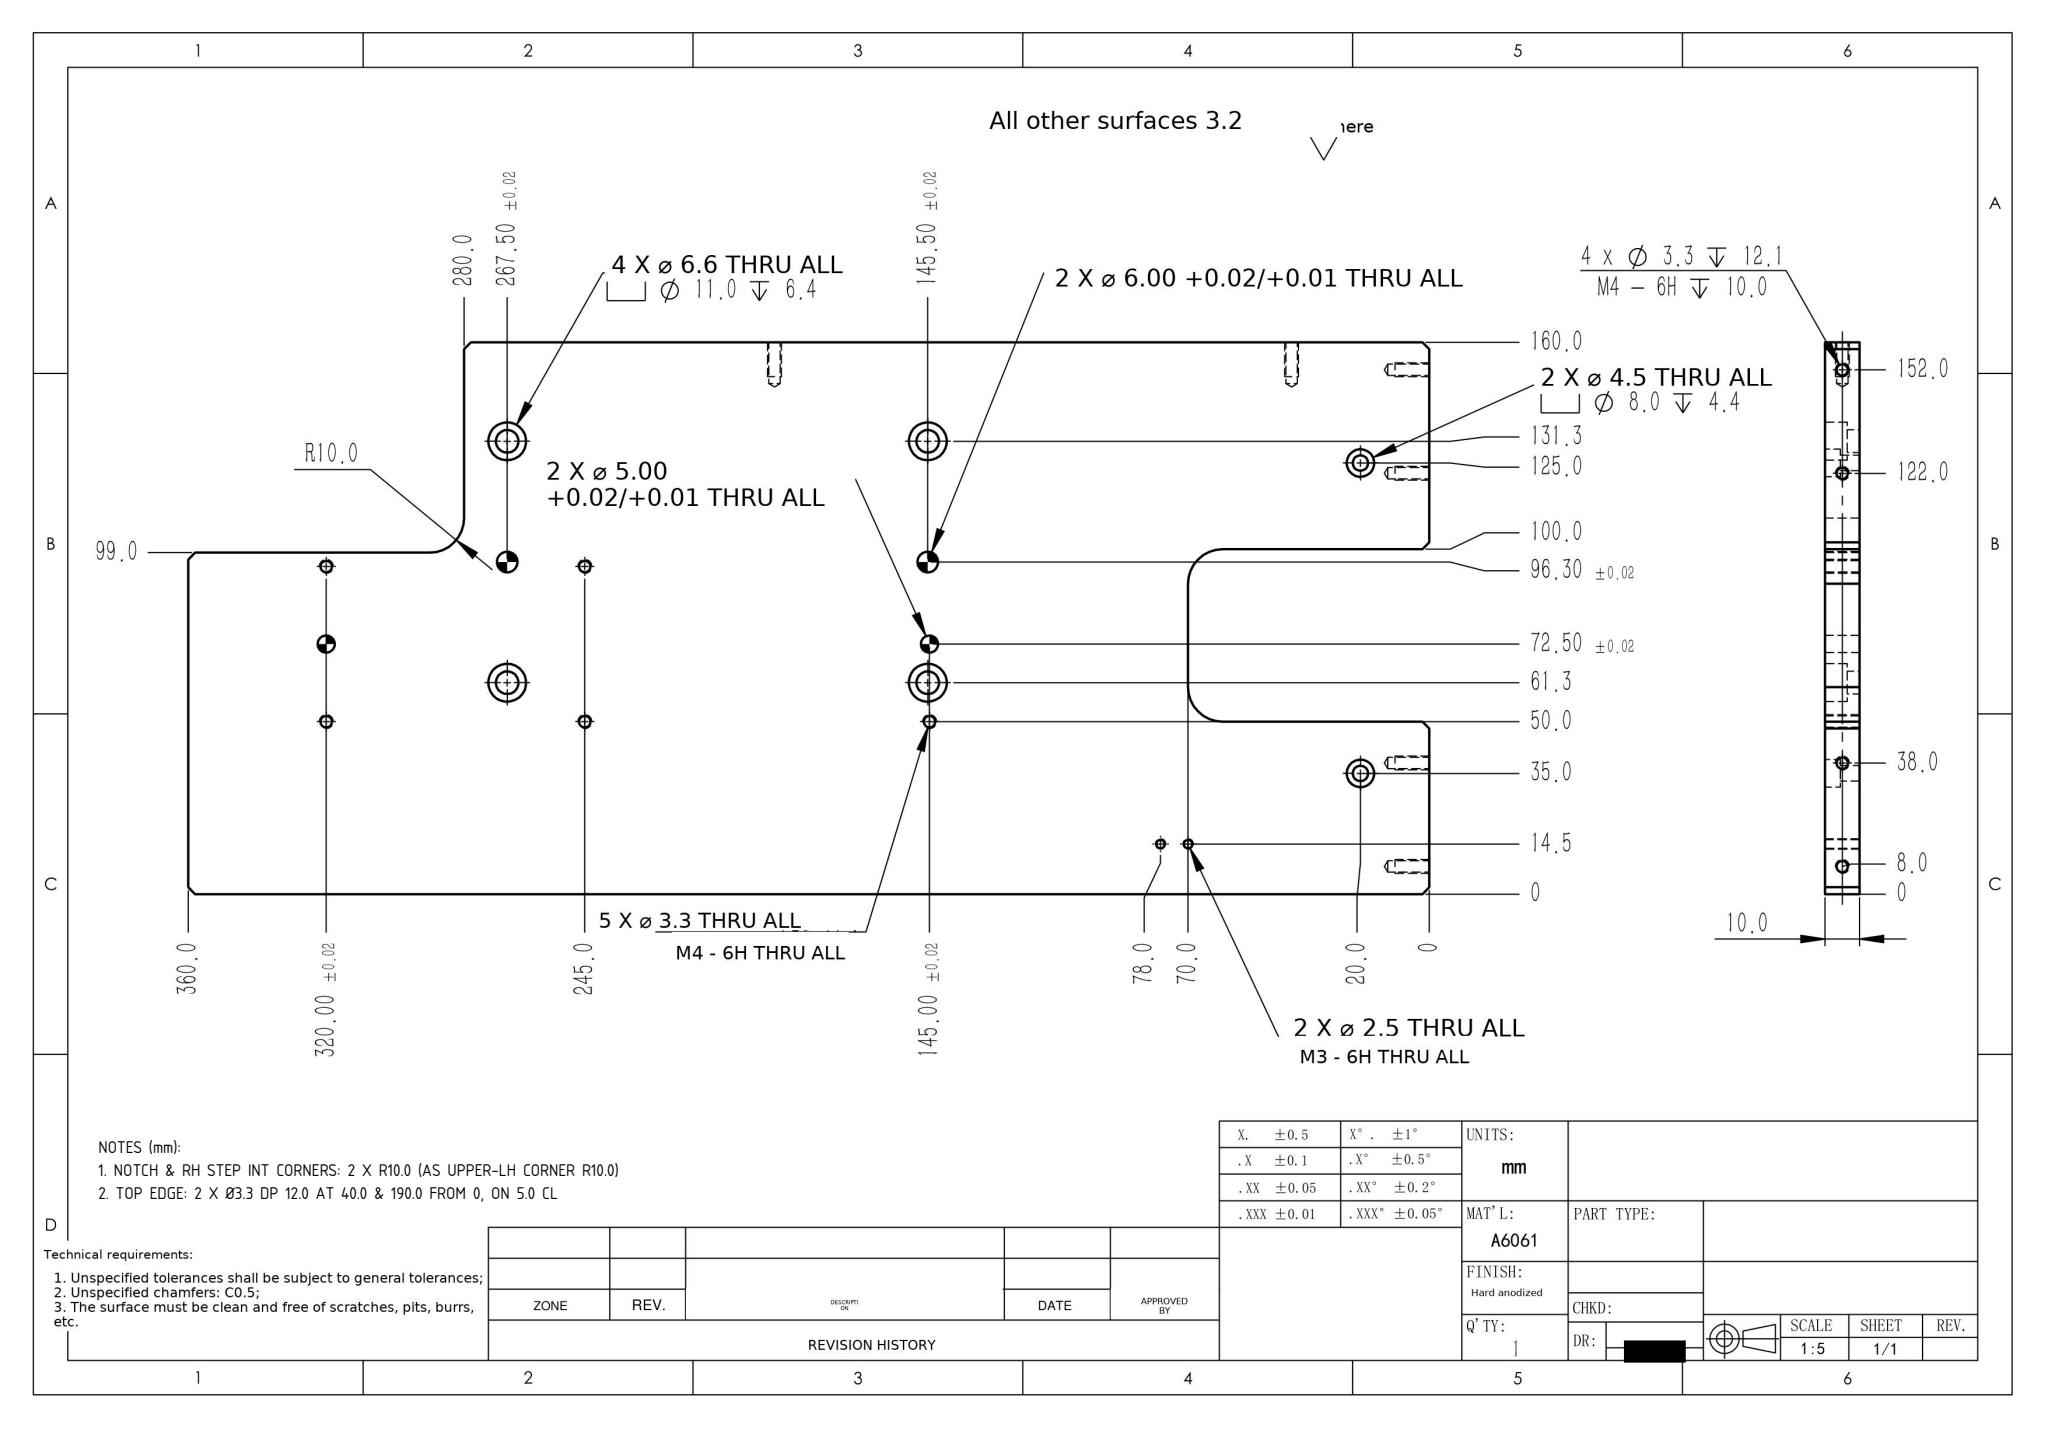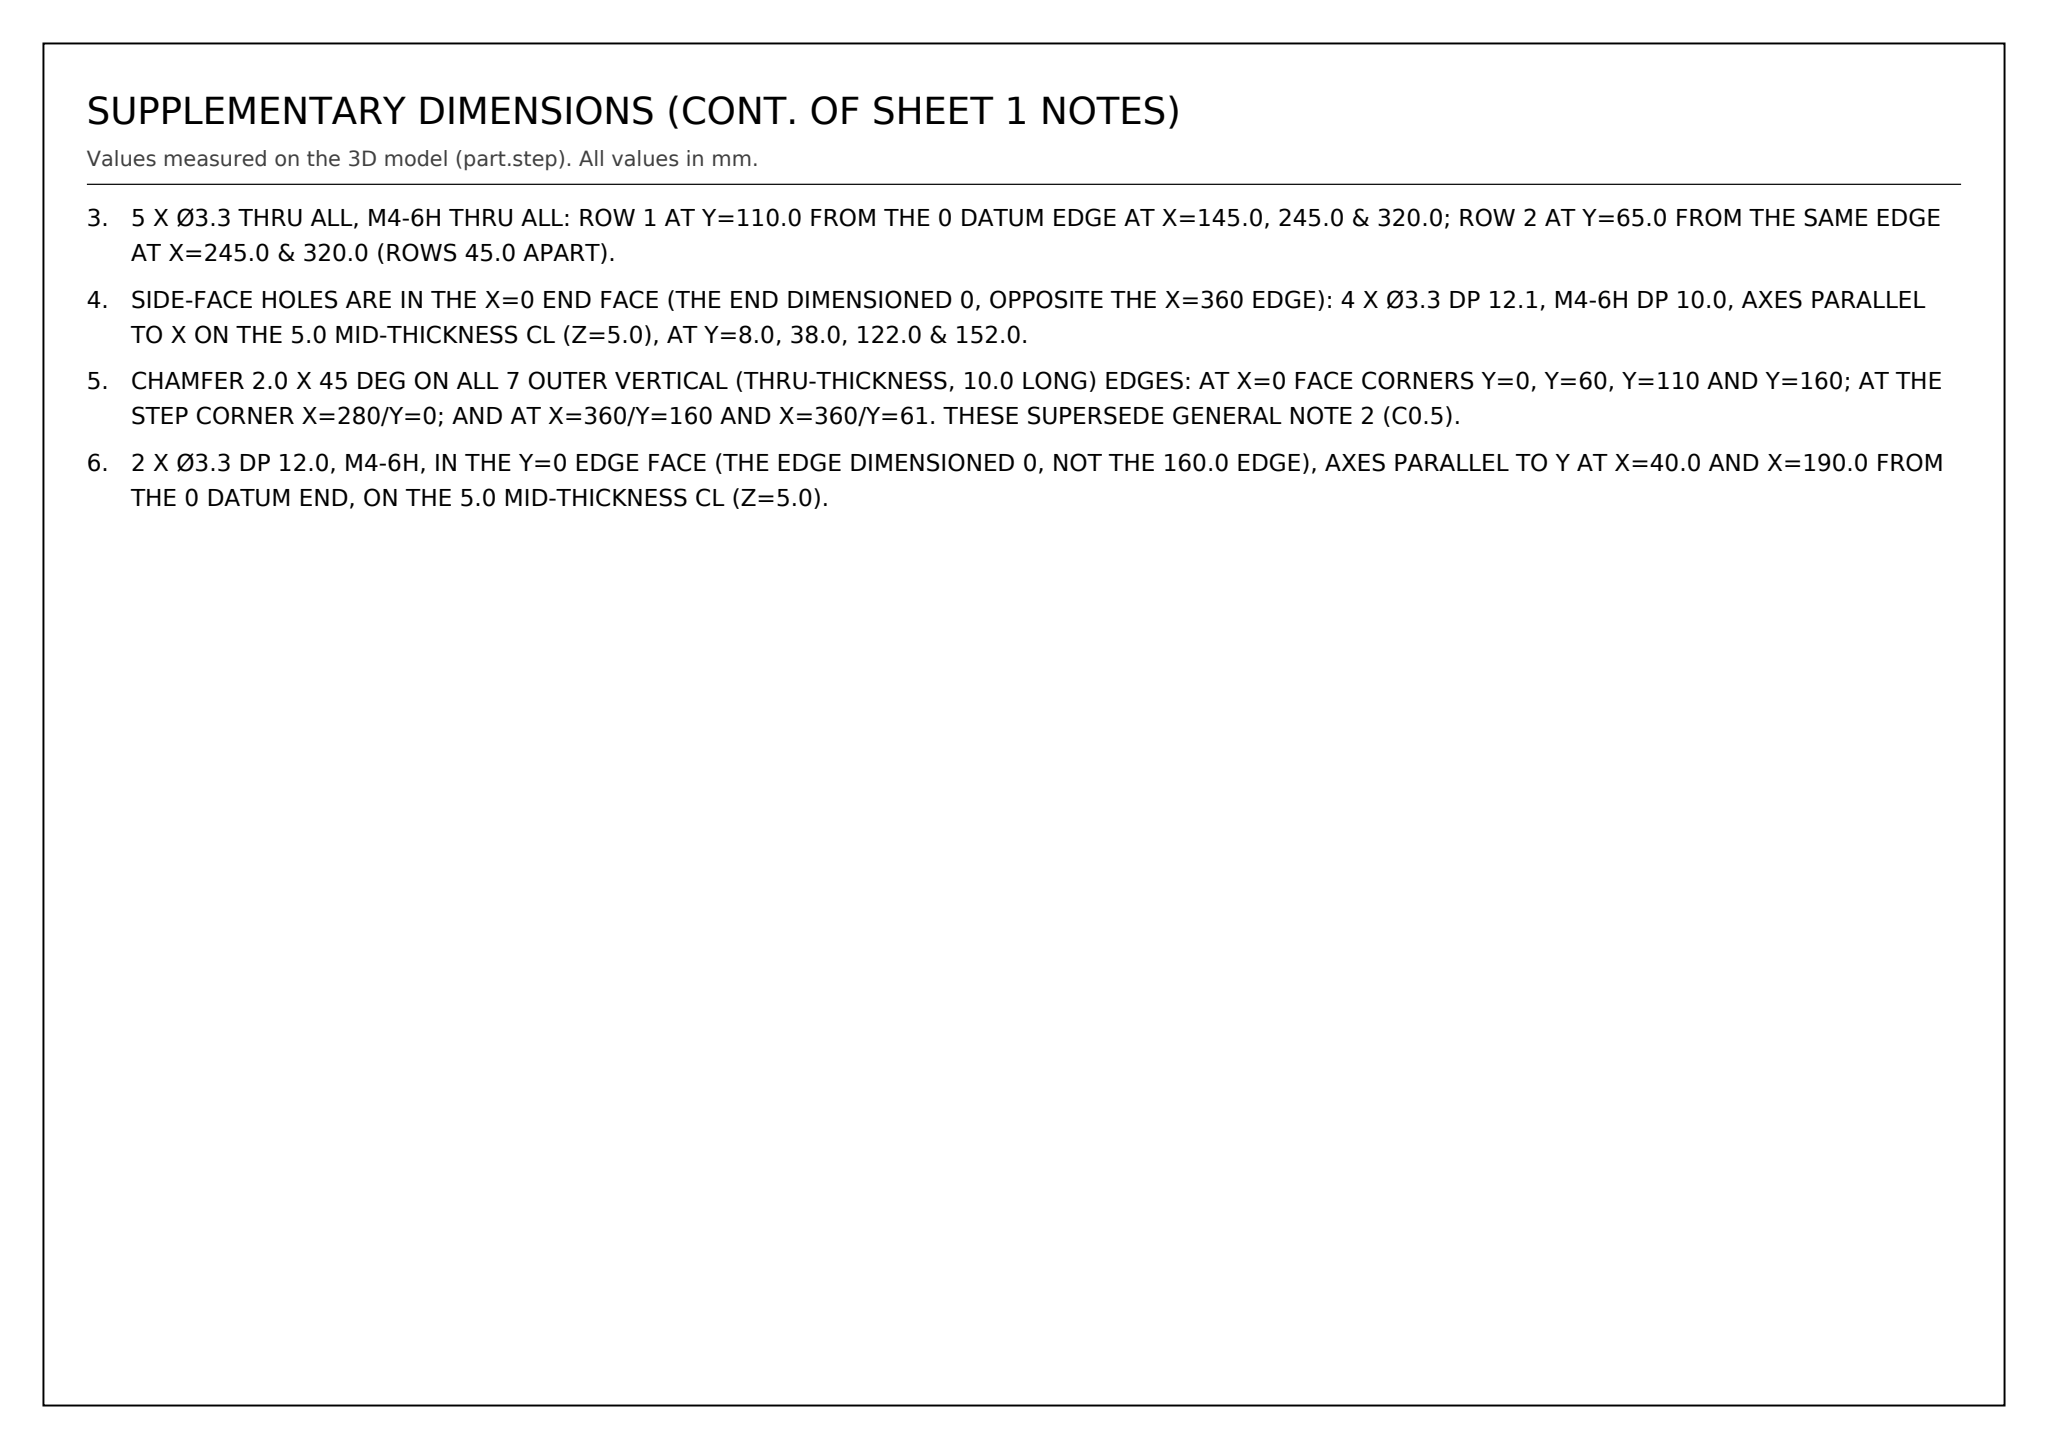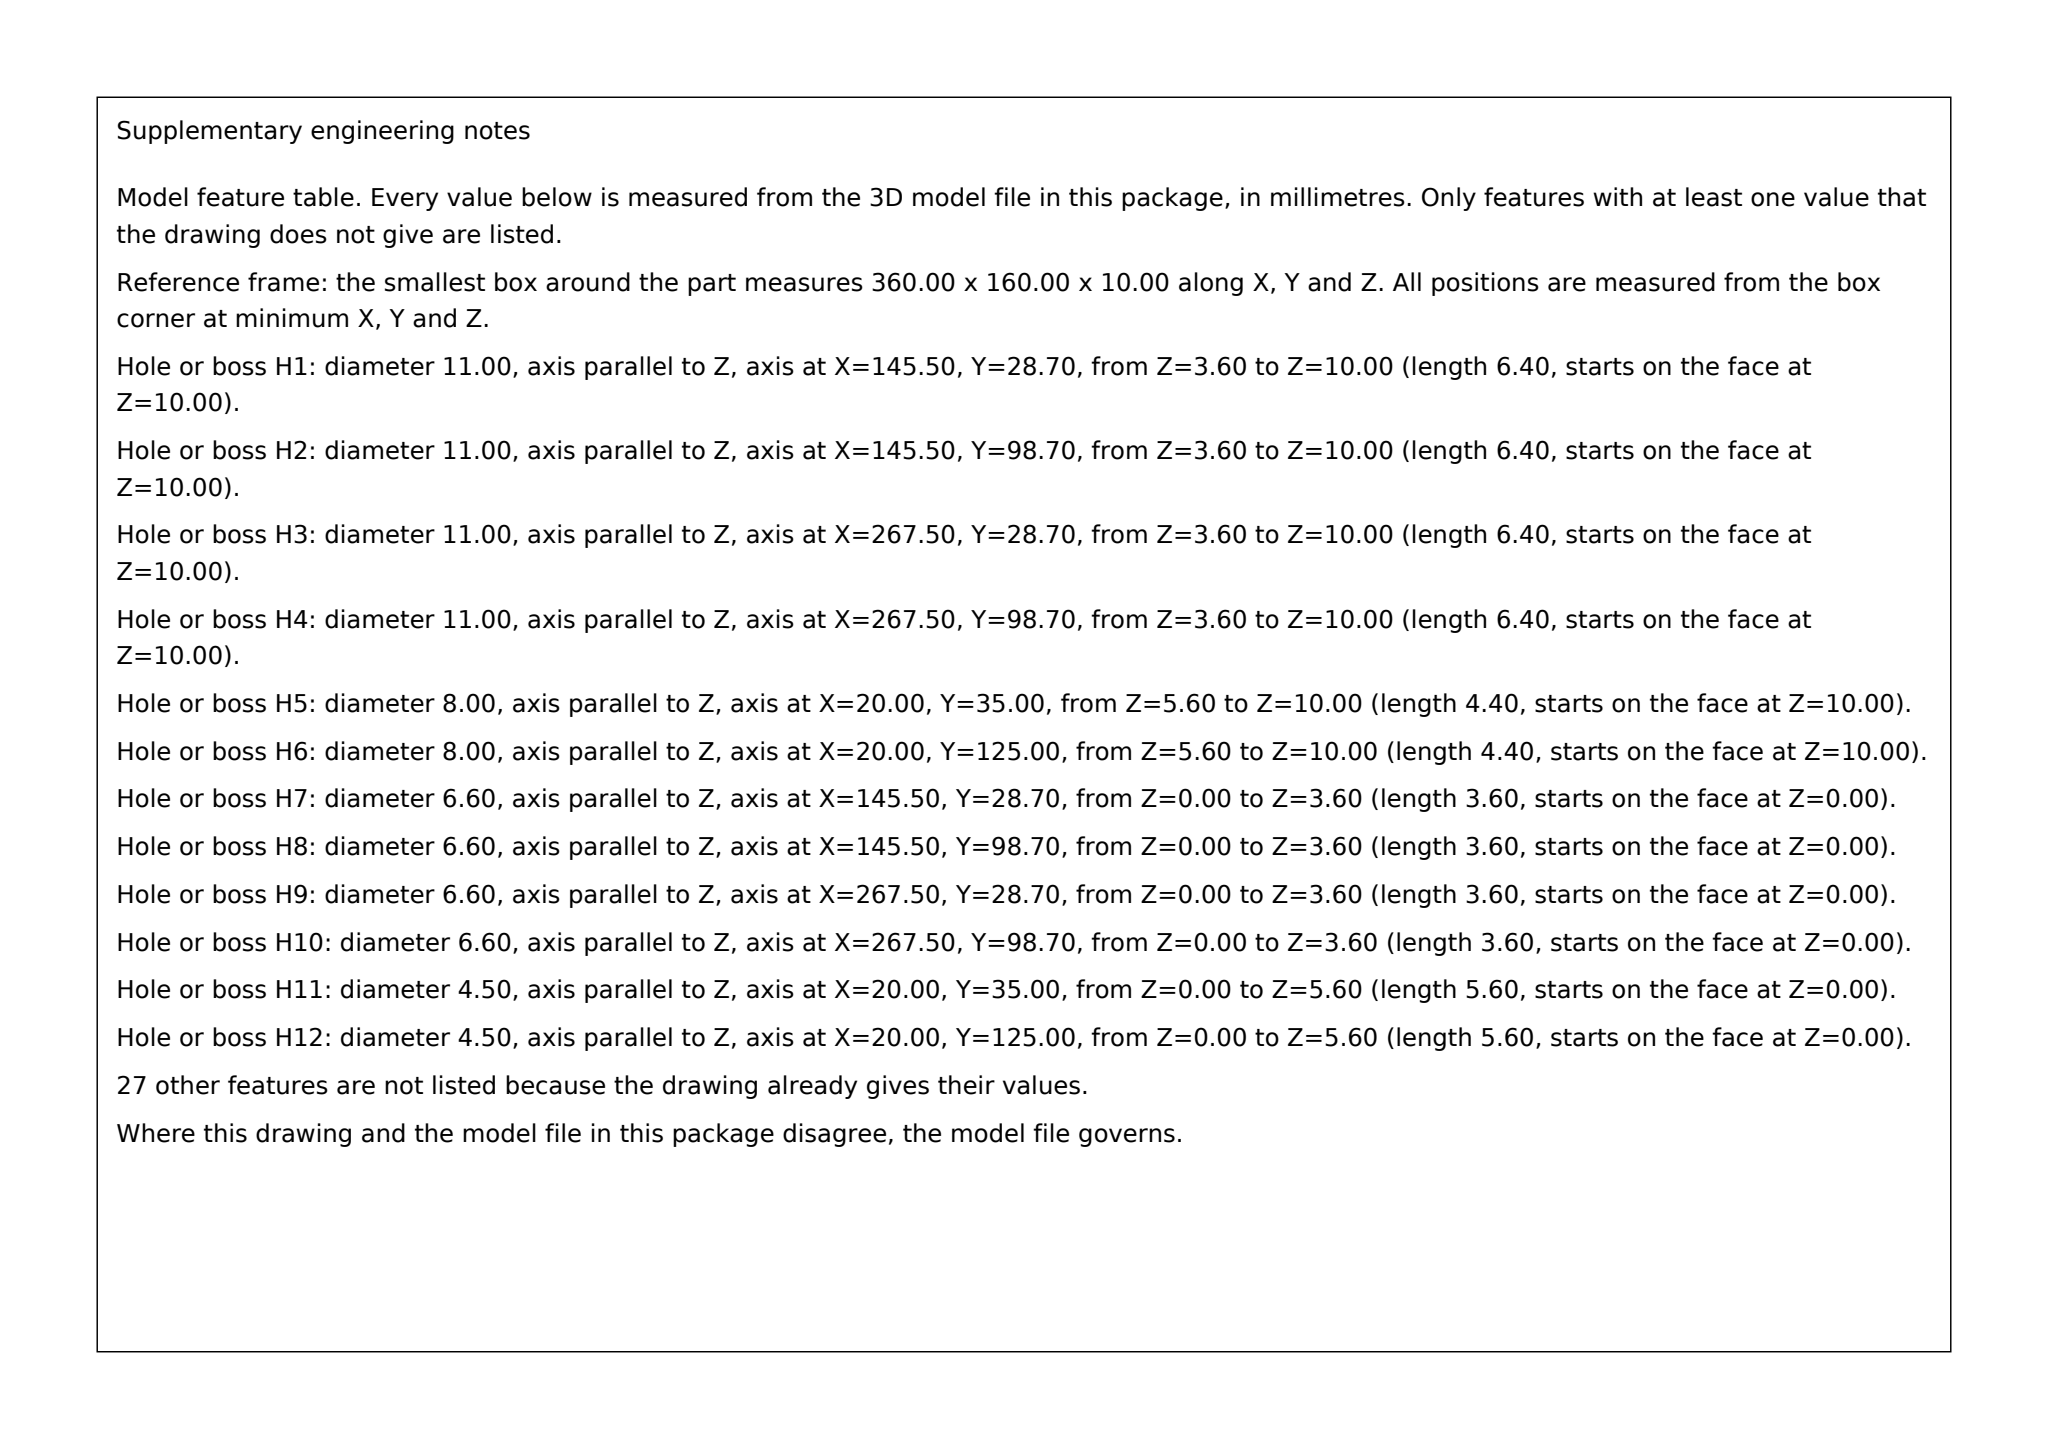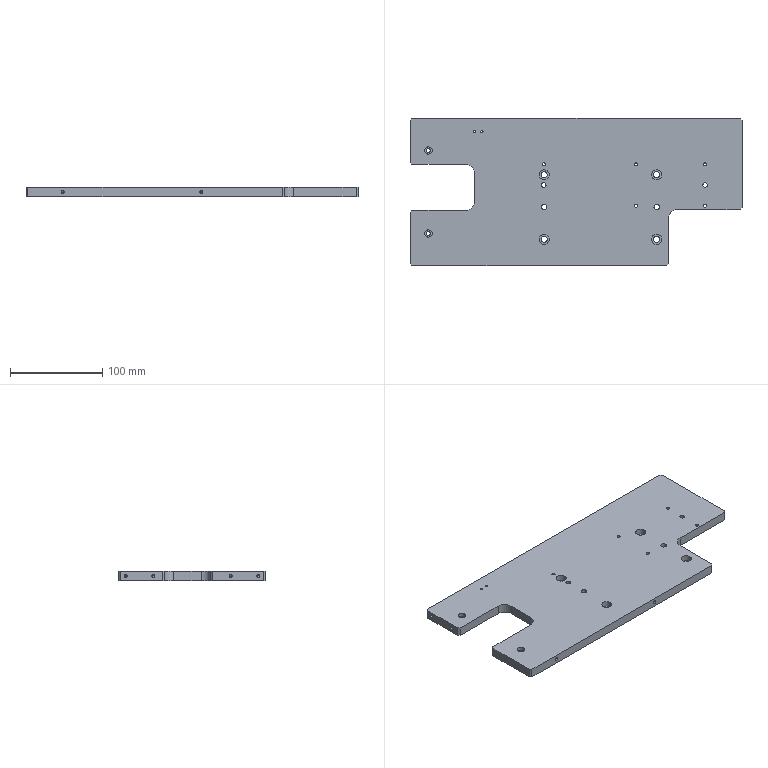Part | SolidWorks | mm | 1 solid | 98 faces | box 360 x 160 x 10 mm | volume 487038 mm3 | cylinder 61 | plane 25 | cone 12 | commonest cylinder face diameters 3.3 x22 11 x8 6.6 x8 8 x4 4.5 x4 5 x4 6 x4 2.5 x4
Drawing notes:
NOTCH & RH STEP INT CORNERS: 2 X R10.0 (AS UPPER-LH CORNER R10.0) | from the solid: Ø20 z-cyls at (60,70) & (60,100) = R10 arcs on planes x=70, y=60 & y=110; same as Ø20 at (290,51) = shown R10.0
TOP EDGE: 2 X Ø3.3 DP 12.0 AT 40.0 & 190.0 FROM 0, ON 5.0 CL | from the solid: Ø3.3 y-axis cyls at [40,-,5.0] & [190,-,5.0], L=12.0, from y=0 face, z=5.0 = mid of 10.0 thk
5 X Ø3.3 THRU ALL, M4-6H THRU ALL: ROW 1 AT Y=110.0 FROM THE 0 DATUM EDGE AT X=145.0, 245.0 & 320.0; ROW 2 AT Y=65.0 FROM THE SAME EDGE AT X=245.0 & 320.0 (ROWS 45.0 APART). | from the solid: cylinders dia 3.3 axis z at (145.0,110.0), (245.0,110.0), (320.0,110.0), (245.0,65.0), (320.0,65.0), from z=0 to 10 (thru 10.0 plate)
SIDE-FACE HOLES ARE IN THE X=0 END FACE (THE END DIMENSIONED 0, OPPOSITE THE X=360 EDGE): 4 X Ø3.3 DP 12.1, M4-6H DP 10.0, AXES PARALLEL TO X ON THE 5.0 MID-THICKNESS CL (Z=5.0), AT Y=8.0, 38.0, 122.0 & 152.0. | from the solid: cylinders dia 3.3 axis x at y=8.0/38.0/122.0/152.0, z=5.0, from x=0.0 to 12.1; planes with normal x at offset 0.0 (y 2-58 and y 112-158)
CHAMFER 2.0 X 45 DEG ON ALL 7 OUTER VERTICAL (THRU-THICKNESS, 10.0 LONG) EDGES: AT X=0 FACE CORNERS Y=0, Y=60, Y=110 AND Y=160; AT THE STEP CORNER X=280/Y=0; AND AT X=360/Y=160 AND X=360/Y=61. THESE SUPERSEDE GENERAL NOTE 2 (C0.5). | from the solid: inclined_planes(chamfers): 7 x 45/45/90 faces, size 2.0 x 2.0 x 10.0, bbox_from [0,0,0], [0,58,0], [0,110,0], [0,158,0], [278,0,0], [358,61,0], [358,158,0]
2 X Ø3.3 DP 12.0, M4-6H, IN THE Y=0 EDGE FACE (THE EDGE DIMENSIONED 0, NOT THE 160.0 EDGE), AXES PARALLEL TO Y AT X=40.0 AND X=190.0 FROM THE 0 DATUM END, ON THE 5.0 MID-THICKNESS CL (Z=5.0). | from the solid: cylinders: hole/bore 3.3 axis y at [40.0,null,5.0] and [190.0,null,5.0], from 0.0 to 12.0; cones 118 deg drill points at y=12.0
build123d program:
from build123d import *

# Parameters (mm, degrees)
SKETCH1_W                                       = 360
SKETCH1_H                                       = 160
BOSS_EXTRUDE1_DEPTH                             = 10
M6_HEX_SOCKET_HEAD_CAP_SCREW_CBORE1_D           = 6.6
M6_HEX_SOCKET_HEAD_CAP_SCREW_CBORE1_CBORE_D     = 11
M6_HEX_SOCKET_HEAD_CAP_SCREW_CBORE1_CBORE_DEPTH = 6.4
M4_TAPPED_HOLE1_D                               = 3.3
M4_TAPPED_HOLE1_DEPTH                           = 12.1
M4_TAPPED_HOLE1_TIP                             = 0.9914
M3_TAPPED_HOLE1_D                               = 2.5
M4_TAPPED_HOLE2_D                               = 3.3
SIZE_MM_DOWEL_PIN_HOLE_1_D                      = 6
SKETCH12_W                                      = 80
SKETCH12_H                                      = 61
CUT_EXTRUDE1_DEPTH                              = 198.231
SIZE_MM_DOWEL_PIN_HOLE_2_D                      = 5
CUT_EXTRUDE2_DEPTH                              = 198.231
CUT_EXTRUDE2_DEPTH_BACK                         = 198.231
SKETCH15_W                                      = 70
SKETCH15_H                                      = 50
M4_TAPPED_HOLE3_D                               = 3.3
M4_TAPPED_HOLE3_DEPTH                           = 12
M4_TAPPED_HOLE3_TIP                             = 0.9914
M4_HEX_SOCKET_HEAD_CAP_SCREW_CBORE1_D           = 4.5
M4_HEX_SOCKET_HEAD_CAP_SCREW_CBORE1_CBORE_D     = 8
M4_HEX_SOCKET_HEAD_CAP_SCREW_CBORE1_CBORE_DEPTH = 4.4
FILLET1_R                                       = 10
CHAMFER1_SIZE                                   = 2


with BuildPart() as part:
    # Sketch1 → Boss-Extrude1 (new body)
    with BuildSketch(Plane.XY):
        Rectangle(SKETCH1_W, SKETCH1_H)
    extrude(amount=BOSS_EXTRUDE1_DEPTH)

    # M6 Hex Socket Head Cap Screw CBORE1 (through all)
    with Locations(Plane.XY.offset(10)):
        with Locations((-34.5, -51.3), (-34.5, 18.7), (87.5, 18.7), (87.5, -51.3)):
            CounterBoreHole(M6_HEX_SOCKET_HEAD_CAP_SCREW_CBORE1_D / 2, M6_HEX_SOCKET_HEAD_CAP_SCREW_CBORE1_CBORE_D / 2, M6_HEX_SOCKET_HEAD_CAP_SCREW_CBORE1_CBORE_DEPTH)

    # M4 Tapped Hole1
    with Locations(Plane.ZY.offset(180)):
        with Locations((5, 42), (5, -42), (5, -72), (5, 72)):
            Hole(M4_TAPPED_HOLE1_D / 2, depth=M4_TAPPED_HOLE1_DEPTH)
            with Locations((0, 0, -(M4_TAPPED_HOLE1_DEPTH + M4_TAPPED_HOLE1_TIP / 2))):  # 118° drill point
                Cone(0, M4_TAPPED_HOLE1_D / 2, M4_TAPPED_HOLE1_TIP, mode=Mode.SUBTRACT)

    # M3 Tapped Hole1 (through all)
    with Locations(Plane.XY.offset(10)):
        with Locations((-110, 65.5), (-102, 65.5)):
            Hole(M3_TAPPED_HOLE1_D / 2)

    # M4 Tapped Hole2 (through all)
    with Locations(Plane.XY.offset(10)):
        with Locations((-35, 30), (65, 30), (140, 30), (140, -15), (65, -15)):
            Hole(M4_TAPPED_HOLE2_D / 2)

    # Size mm Dowel Pin Hole 1 (through all)
    with Locations(Plane.XY.offset(10)):
        with Locations((-34.5, -16.3), (87.5, -16.3)):
            Hole(SIZE_MM_DOWEL_PIN_HOLE_1_D / 2)

    # Sketch12 → Cut-Extrude1 (cut, through all)
    with BuildSketch(Plane.XY.offset(10)):
        with Locations((140, -49.5)):
            Rectangle(SKETCH12_W, SKETCH12_H)
    extrude(amount=-CUT_EXTRUDE1_DEPTH, mode=Mode.SUBTRACT)

    # Size mm Dowel Pin Hole 2 (through all)
    with Locations(Plane.XY.offset(10)):
        with Locations((-35, 7.5), (140, 7.5)):
            Hole(SIZE_MM_DOWEL_PIN_HOLE_2_D / 2)

    # Sketch15 → Cut-Extrude2 (cut, two sides: drawn at the far end of the back side and taken through both)
    with BuildSketch(Plane.XY.offset(10).offset(-CUT_EXTRUDE2_DEPTH_BACK)):
        with Locations((-145, 5)):
            Rectangle(SKETCH15_W, SKETCH15_H)
    extrude(amount=CUT_EXTRUDE2_DEPTH + CUT_EXTRUDE2_DEPTH_BACK, mode=Mode.SUBTRACT)

    # M4 Tapped Hole3
    with Locations(Plane(origin=(0, -80, 0), x_dir=(-1, 0, 0), z_dir=(0, -1, 0))):
        with Locations((140, -5), (-10, -5)):
            Hole(M4_TAPPED_HOLE3_D / 2, depth=M4_TAPPED_HOLE3_DEPTH)
            with Locations((0, 0, -(M4_TAPPED_HOLE3_DEPTH + M4_TAPPED_HOLE3_TIP / 2))):  # 118° drill point
                Cone(0, M4_TAPPED_HOLE3_D / 2, M4_TAPPED_HOLE3_TIP, mode=Mode.SUBTRACT)

    # M4 Hex Socket Head Cap Screw CBORE1 (through all)
    with Locations(Plane.XY.offset(10)):
        with Locations((-160, -45), (-160, 45)):
            CounterBoreHole(M4_HEX_SOCKET_HEAD_CAP_SCREW_CBORE1_D / 2, M4_HEX_SOCKET_HEAD_CAP_SCREW_CBORE1_CBORE_D / 2, M4_HEX_SOCKET_HEAD_CAP_SCREW_CBORE1_CBORE_DEPTH)

    # Fillet1
    fillet1_edges = [part.edges().sort_by_distance(p)[0] for p in [
        (100, -19, 5),
        (-110, 30, 5),
        (-110, -20, 5),
    ]]
    fillet(fillet1_edges, radius=FILLET1_R)

    # Chamfer1
    chamfer1_edges = [part.edges().sort_by_distance(p)[0] for p in [
        (180, -19, 5),
        (100, -80, 5),
        (-180, -20, 5),
        (-180, 30, 5),
        (-180, -80, 5),
        (-180, 80, 5),
        (180, 80, 5),
    ]]
    chamfer(chamfer1_edges, length=CHAMFER1_SIZE)


solid = part.part